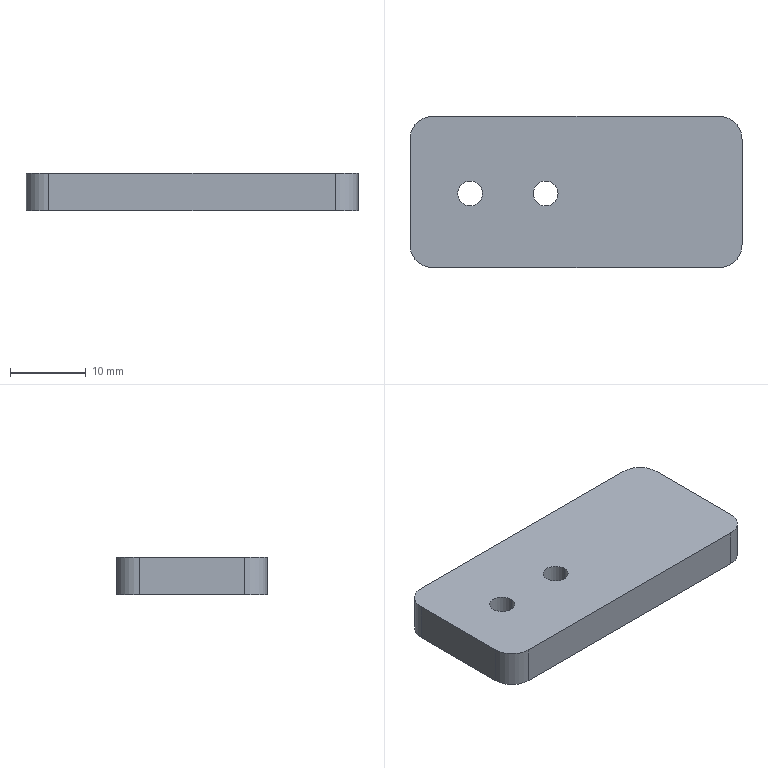Component | SolidWorks | 3UpperBaffle-RearSmallBaffle9.26-1 | 1 solid | 14 faces | box 43.97 x 20 x 5 mm | volume 4273 mm3 | cylinder 8 | plane 6 | commonest cylinder face diameters 3.3 x4 6 x4 | material AISI 1045 Steel, Cold Drawn
build123d program:
from build123d import *

# Parameters (mm, degrees)
BOSS_EXTRUDE1_DEPTH = 5
SKETCH2_W           = 5
SKETCH2_H           = 14
BOSS_EXTRUDE2_DEPTH = 30
SKETCH3_R           = 4
CUT_EXTRUDE1_DEPTH  = 479.713
FILLET1_R           = 4
CUT_EXTRUDE2_DEPTH  = 479.713
FILLET2_R           = 3
M4_TAPPED_HOLE1_D   = 3.3


with BuildPart() as part:
    # Sketch1 → Boss-Extrude1 (new body)
    with BuildSketch(Plane.XY):
        Polygon((0, 0), (30, 0), (425.189, 84), (471.259, 84), (471.259, 64), (427.291, 64), (32.102, -20), (0, -20), align=None)
    extrude(amount=BOSS_EXTRUDE1_DEPTH)

    # Sketch2 → Boss-Extrude2 (add)
    with BuildSketch(Plane.ZY):
        with Locations((2.5, -13)):
            Rectangle(SKETCH2_W, SKETCH2_H)
    extrude(amount=BOSS_EXTRUDE2_DEPTH)

    # Sketch3 → Cut-Extrude1 (cut, through all)
    with BuildSketch(Plane.XY.offset(5)):
        with Locations((130, 11.032)):
            Circle(SKETCH3_R)
        with Locations((170, 19.535)):
            Circle(SKETCH3_R)
        with Locations((266, 39.94)):
            Circle(SKETCH3_R)
        with Locations((306, 48.442)):
            Circle(SKETCH3_R)
    extrude(amount=-CUT_EXTRUDE1_DEPTH, mode=Mode.SUBTRACT)

    # Fillet1
    fillet1_edges = [part.edges().sort_by_distance(p)[0] for p in [
        (-30, -6, 2.5),
        (0, 0, 2.5),
    ]]
    fillet(fillet1_edges, radius=FILLET1_R)

    # Sketch4 → Cut-Extrude2 (cut, through all)
    with BuildSketch(Plane.XY.offset(5)):
        Polygon((427.291, 64), (427.291, -279.86), (-65.05, -270.347), (-65.05, 163.199), (420.125, 114.269), (427.291, 114.269), align=None)
    extrude(amount=-CUT_EXTRUDE2_DEPTH, mode=Mode.SUBTRACT)

    # Fillet2
    fillet2_edges = [part.edges().sort_by_distance(p)[0] for p in [
        (471.259, 84, 2.5),
        (471.259, 64, 2.5),
        (427.291, 64, 2.5),
        (427.291, 84, 2.5),
    ]]
    fillet(fillet2_edges, radius=FILLET2_R)

    # M4 Tapped Hole1 (through all)
    with Locations(Plane.XY.offset(5)):
        with Locations((445.259, 73.799), (435.259, 73.799)):
            Hole(M4_TAPPED_HOLE1_D / 2)


solid = part.part

# Placed as in the assembly
solid = solid.moved(Location((-30, 41.165, 12.75), (0, 0, 0)))